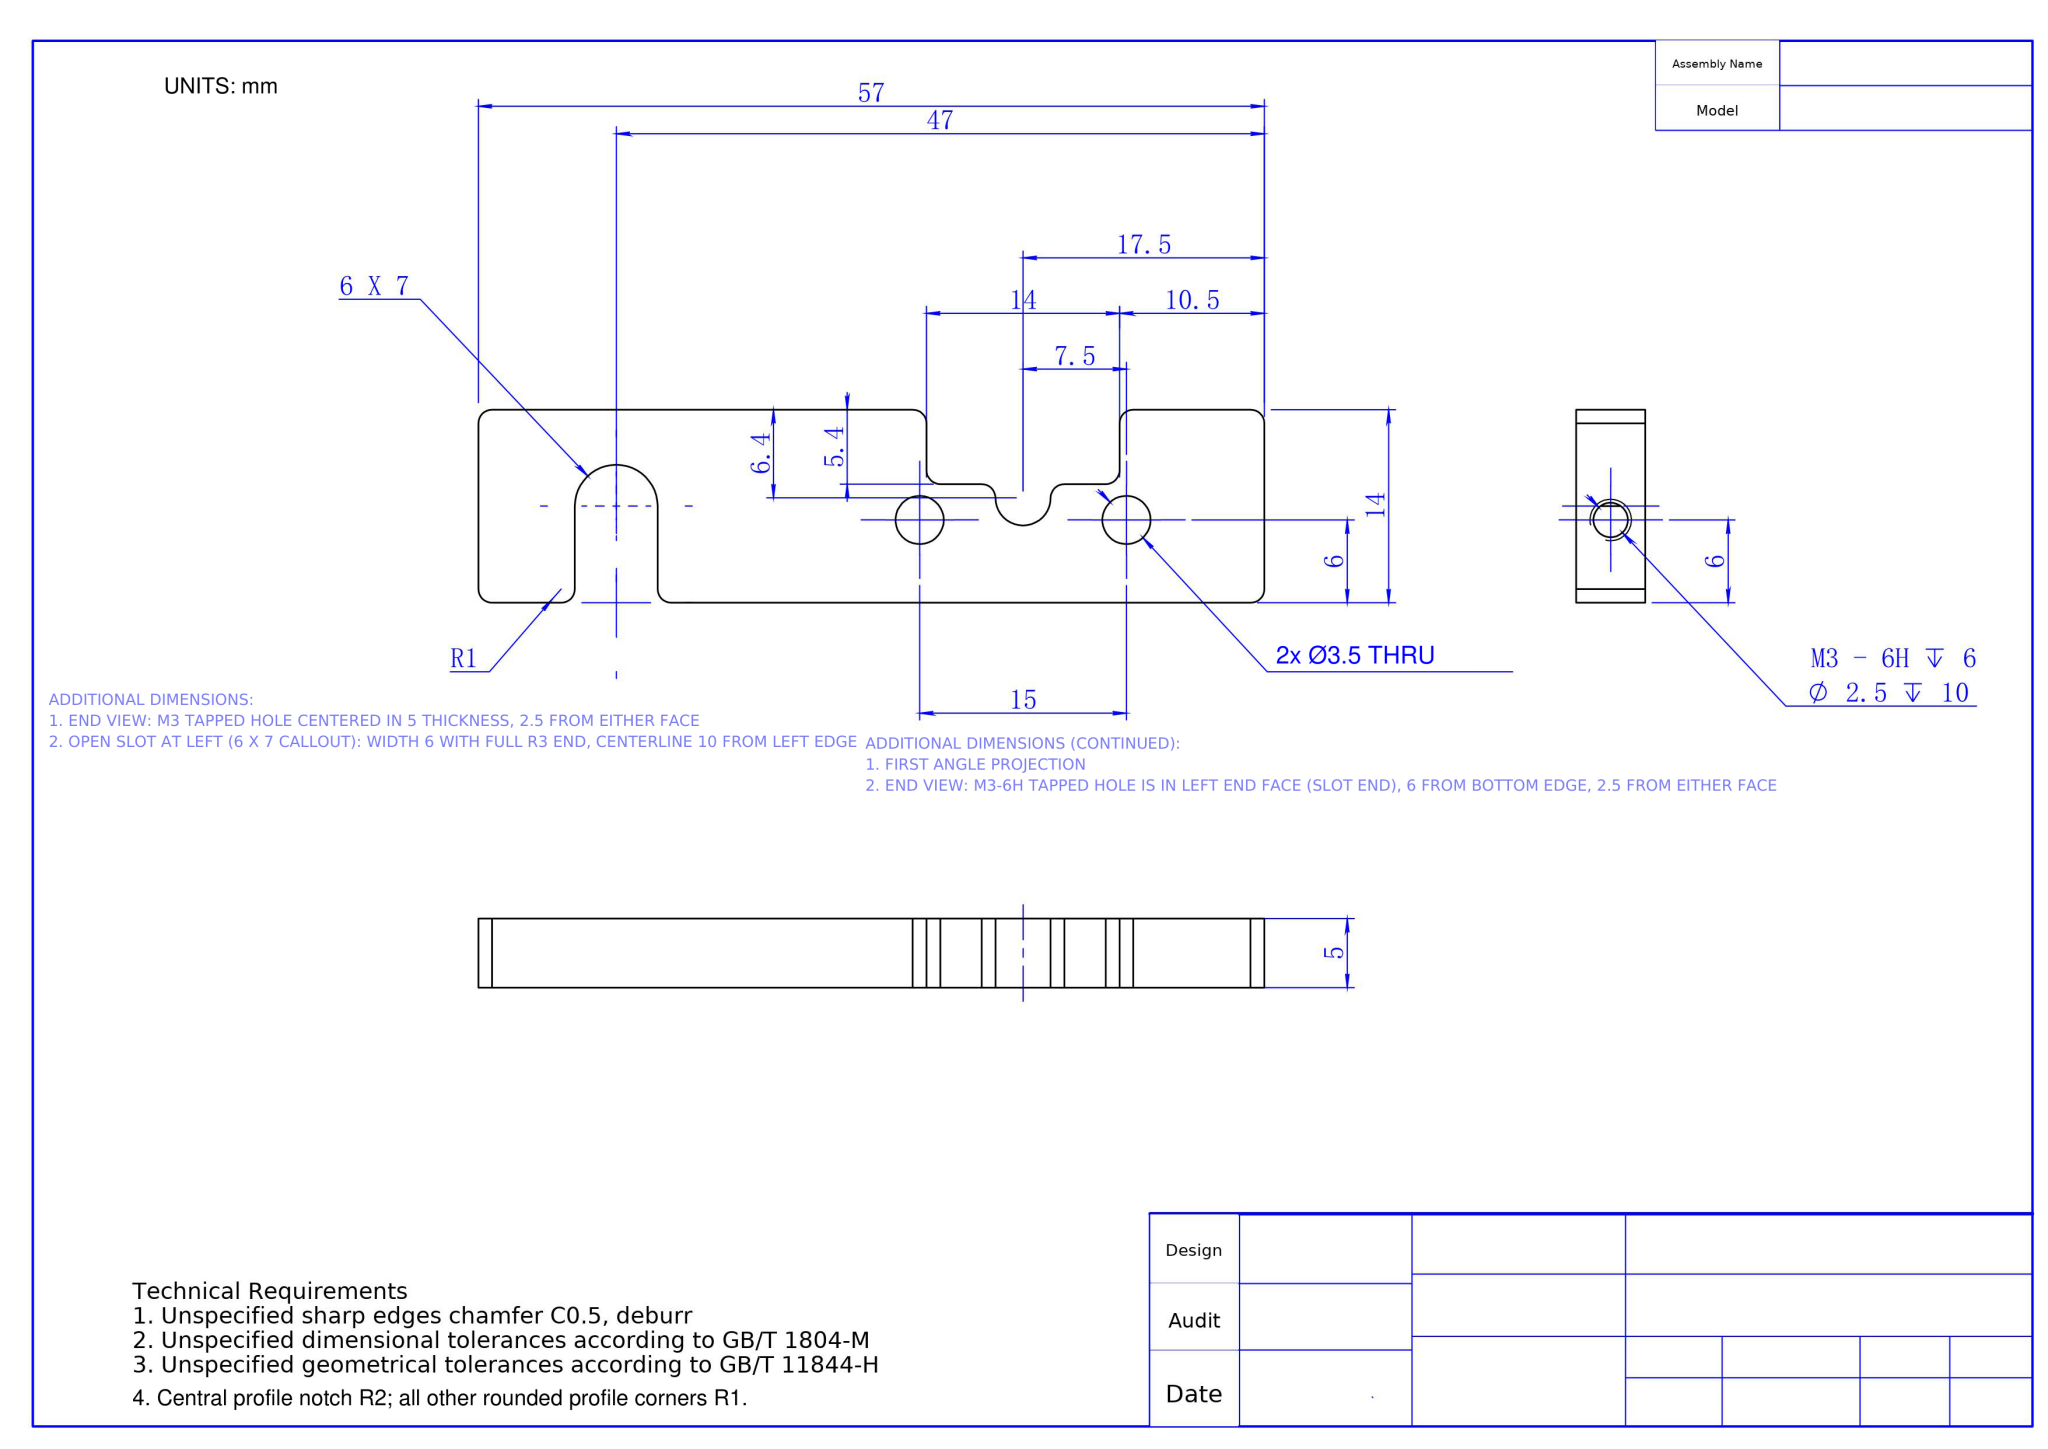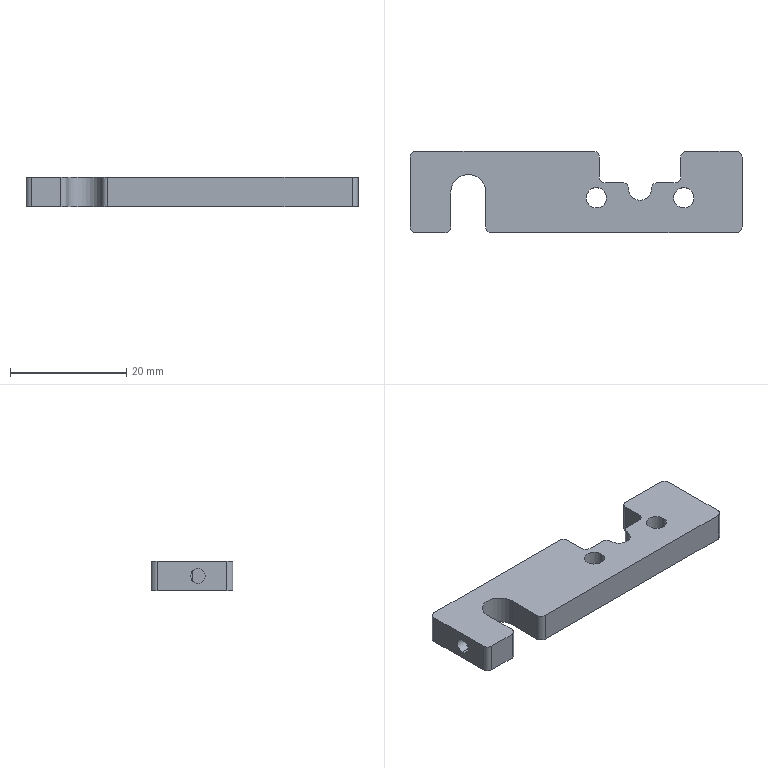Part | NX | mm | 1 solid | 34 faces | box 57 x 14 x 5 mm | volume 3141 mm3 | cylinder 20 | plane 14 | commonest cylinder face diameters 2 x12 3.5 x4 2.5 x2 6 x1 4 x1